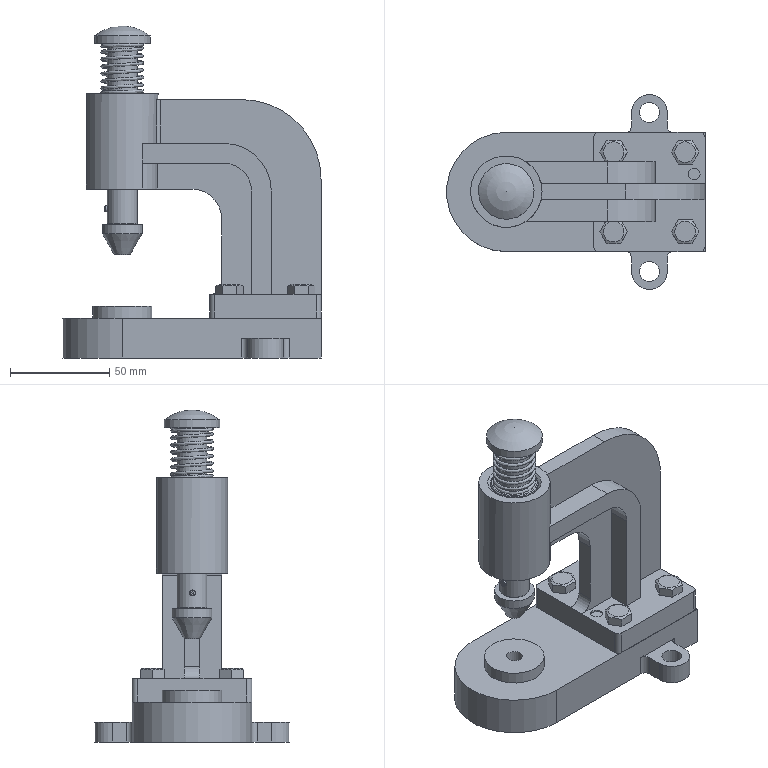Assembly | NX | mm | 14 component files | 14 solids | 181 faces | box 130 x 98 x 167 mm | volume 335801 mm3 | plane 96 | cylinder 56 | cone 23 | spline 5 | sphere 1 | commonest cylinder face diameters 6 x20 5 x4 6.6 x4 28 x3 3 x2 16 x2 30 x2 24 x2
Bill of materials:
unnamed part 1 | 4 |  | Hex-head bolt-like part: hexagonal head with chamfered top edges and a plain cylindrical shank with a chamfered tip.
unnamed part 2 | 1 |  | Flat plate with one rounded end. It has a large hole near the rounded end, several small through holes, and two thinner lugs with holes on opposite sides.
unnamed part 3 | 1 |  | Plain cylindrical tube or sleeve with a concentric through bore and small chamfers on both ends.
unnamed part 4 | 1 |  | Flanged cylindrical part: a wide thin disc flange on a smaller cylindrical body, with a centered axial hole and a chamfer at the end of the body.
unnamed part 5 | 1 |  | Solid cylindrical pin with chamfered ends and a small rectangular notch or flat cut near one end.
unnamed part 6 | 1 |  | L-shaped bracket: a rectangular base plate with mounting holes, an upright that curves over into a horizontal arm, and a ring boss with a bore at the end of the arm.
unnamed part 7 | 1 |  | Helical coil spring made of round wire, with many evenly spaced open coils and flattened, closed end coils.
unnamed part 8 | 1 |  | Rivet- or pin-like part: a low domed round head on a long plain cylindrical shank.
unnamed part 9 | 1 |  | Turned part: a cylindrical disc collar with a cone tapering to a flat end below it and a smaller cylindrical pin on top with a chamfered tip.
unnamed part 10 | 2 |  | Plain solid cylindrical rod with flat ends.
Mates:
1. fix | base 1 component
2. concentric | base 1 arc | bracket 1 arc
3. parallel | bracket 1 face | base 1 face
4. concentric | bushing 1 edge | bracket 1 arc
5. touch align | SPRING_CYLINDER_COMPRESSION_1 1 datumaxis | bushing 1 face
6. touch align | SPRING_CYLINDER_COMPRESSION_1 1 face | bushing 1 face
7. touch align | ram 1 face | bracket 1 face
8. touch align | SPRING_CYLINDER_COMPRESSION_1 1 face | ram 1 face
9. touch align | mold 1 line | ram 1 face
10. touch align | mold 1 face | ram 1 face
11. touch align | pin_A6X30 2 face | bracket 1 face
12. center | pin_A6X30 2 face | pin_A6X30 2 face | base 1 face | bracket 1 face
13. touch align | pin_A6X30 1 face | bracket 1 face
14. center | pin_A6X30 1 face | pin_A6X30 1 face | base 1 face | bracket 1 face
15. concentric | bracket 1 edge | bolt_M6X25 4 edge
16. parallel | bolt_M6X25 4 face | bracket 1 face
17. concentric | bracket 1 edge | bolt_M6X25 3 edge
18. parallel | bolt_M6X25 3 face | bracket 1 face
19. concentric | bracket 1 edge | bolt_M6X25 2 edge
20. parallel | bolt_M6X25 2 face | bracket 1 face
21. concentric | bracket 1 edge | bolt_M6X25 1 edge
22. parallel | bolt_M6X25 1 face | bracket 1 face
23. concentric | base 1 edge | mold_base_assy 1 edge